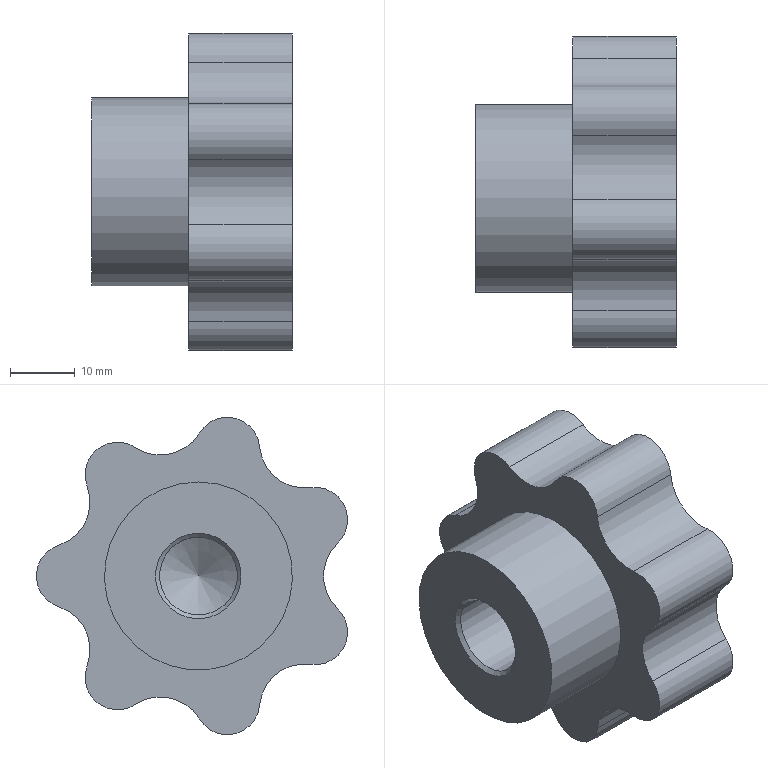Component | NX | THUMB_NUT | 1 solid | 21 faces | volume 31477 mm3 | cylinder 16 | plane 3 | cone 2 | commonest cylinder face diameters 10 x7 14 x7 29 x1 12 x1